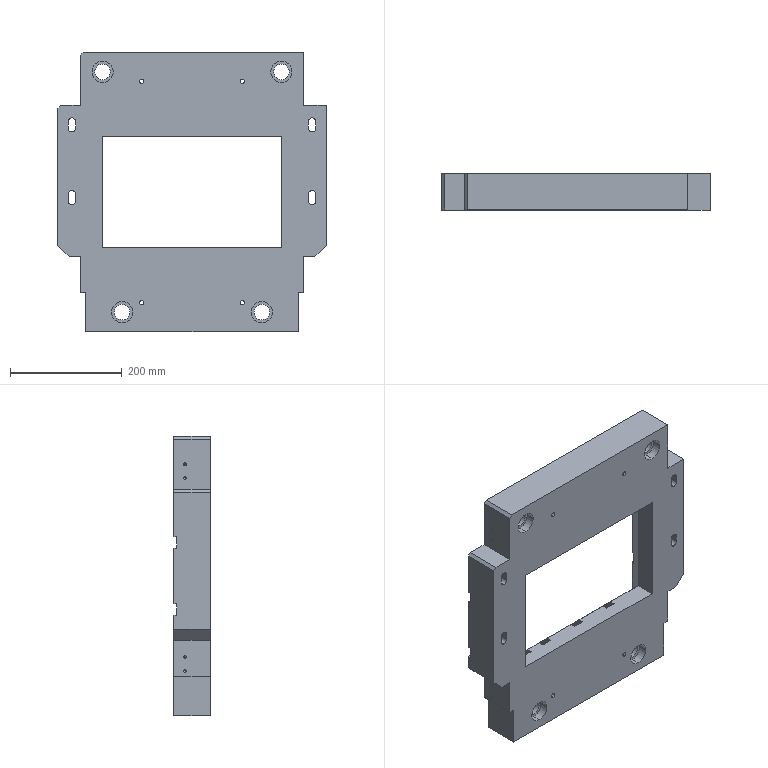Component | SolidWorks | NewDieSet-1_LowerDieSetAssembly-1_LowerDieSet-1 | 1 solid | 213 faces | volume 9141176 mm3 | plane 113 | cylinder 78 | cone 22 | commonest cylinder face diameters 5 x16 38 x16 20 x12 13.5 x12 8 x8 28 x8 10.2 x6